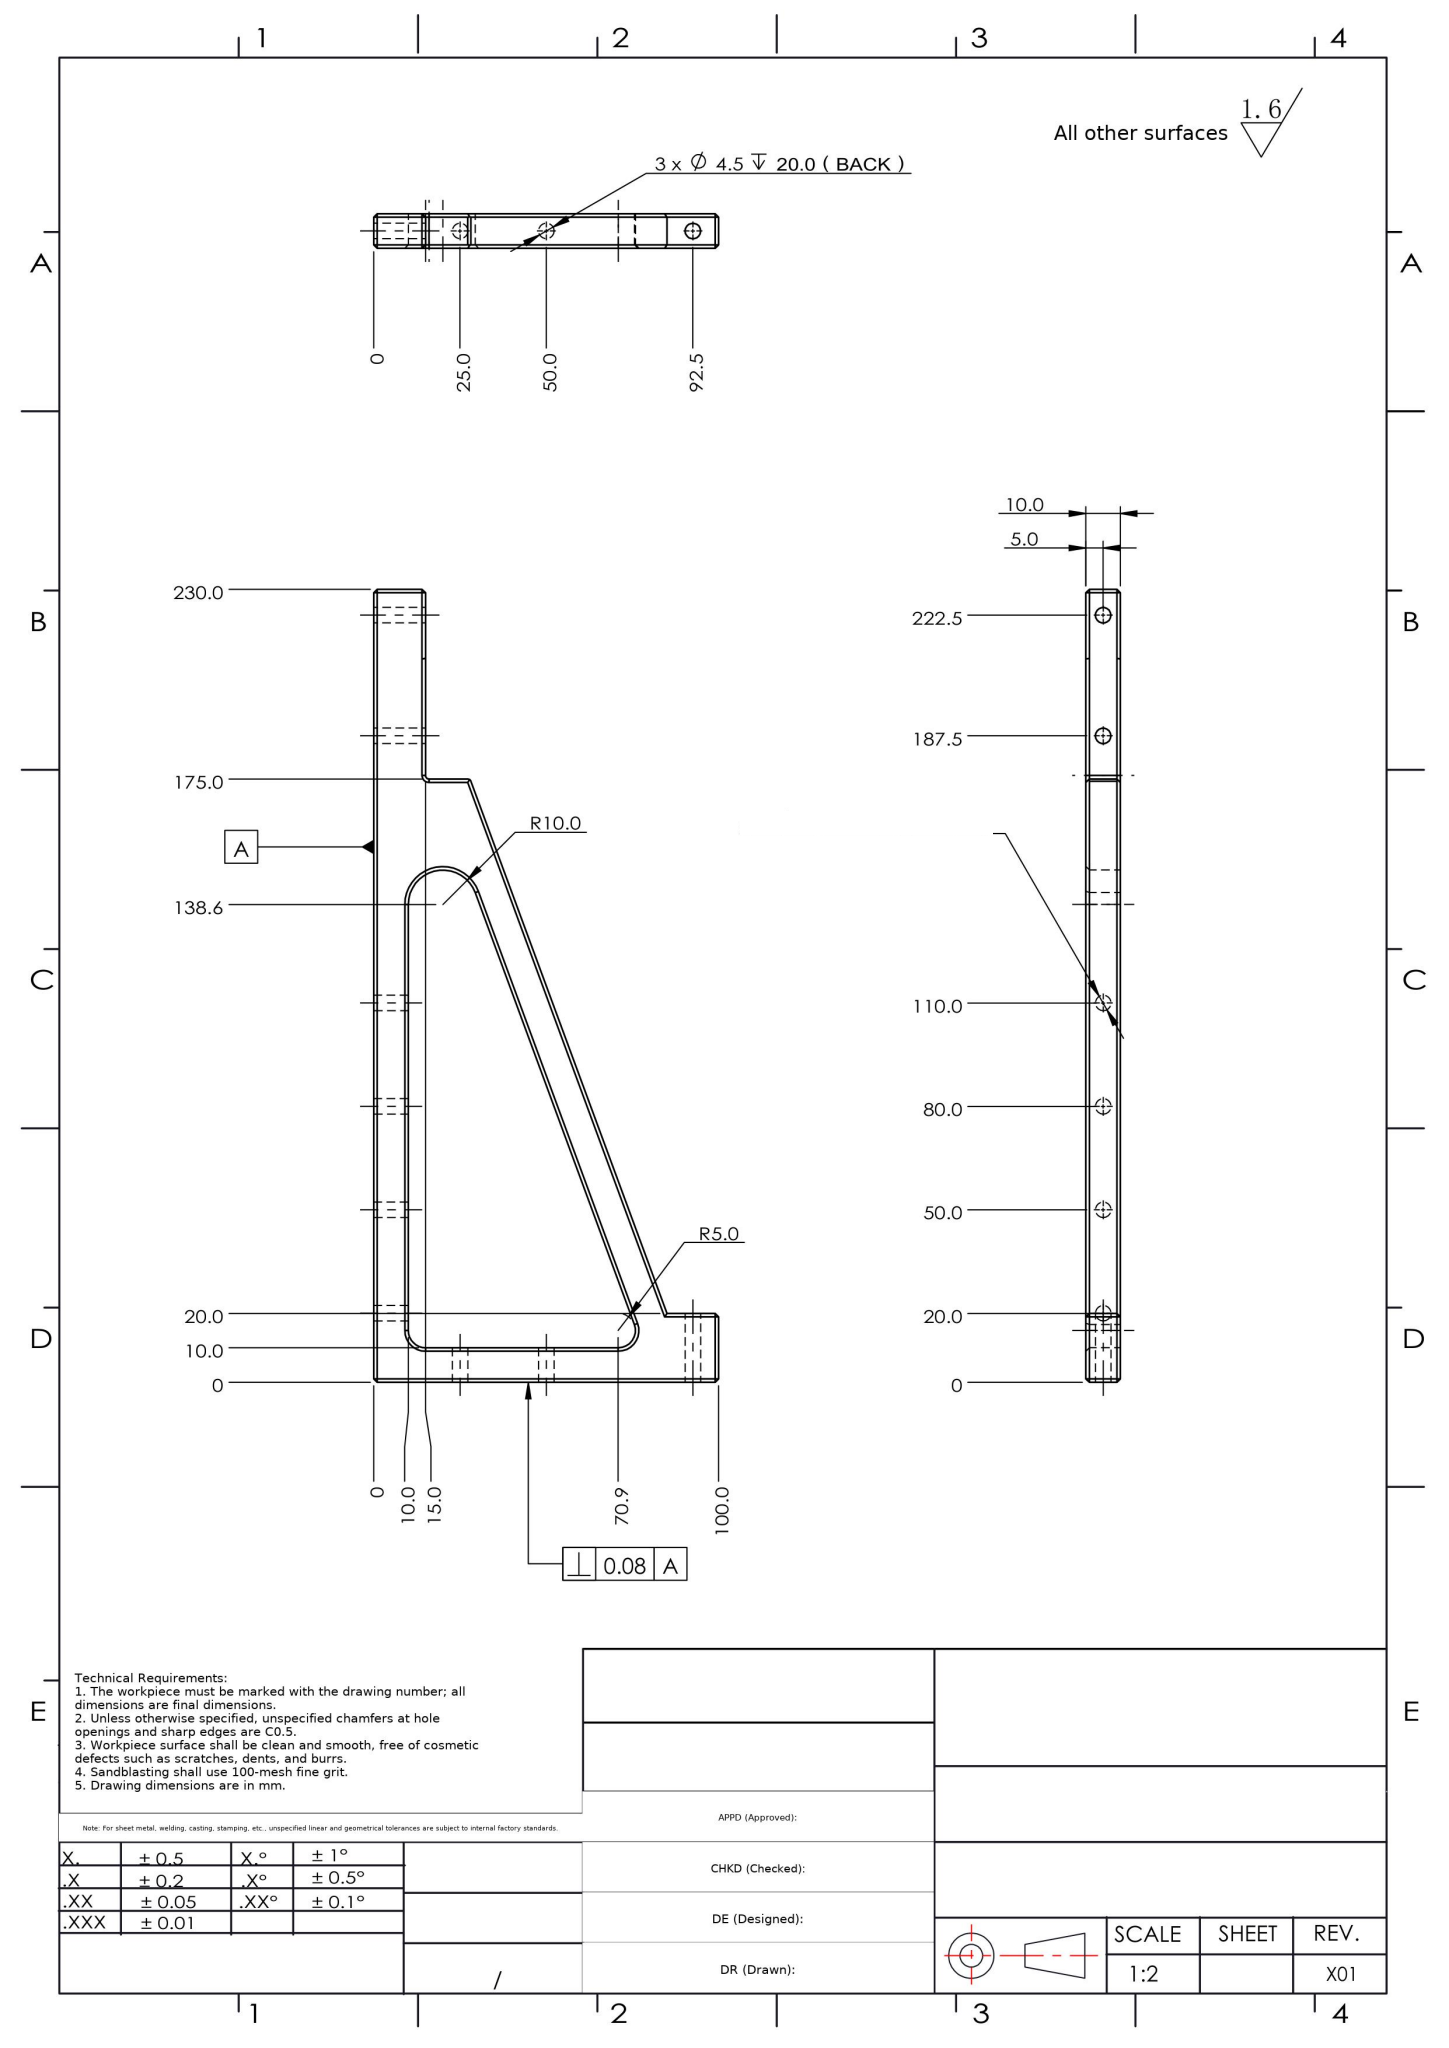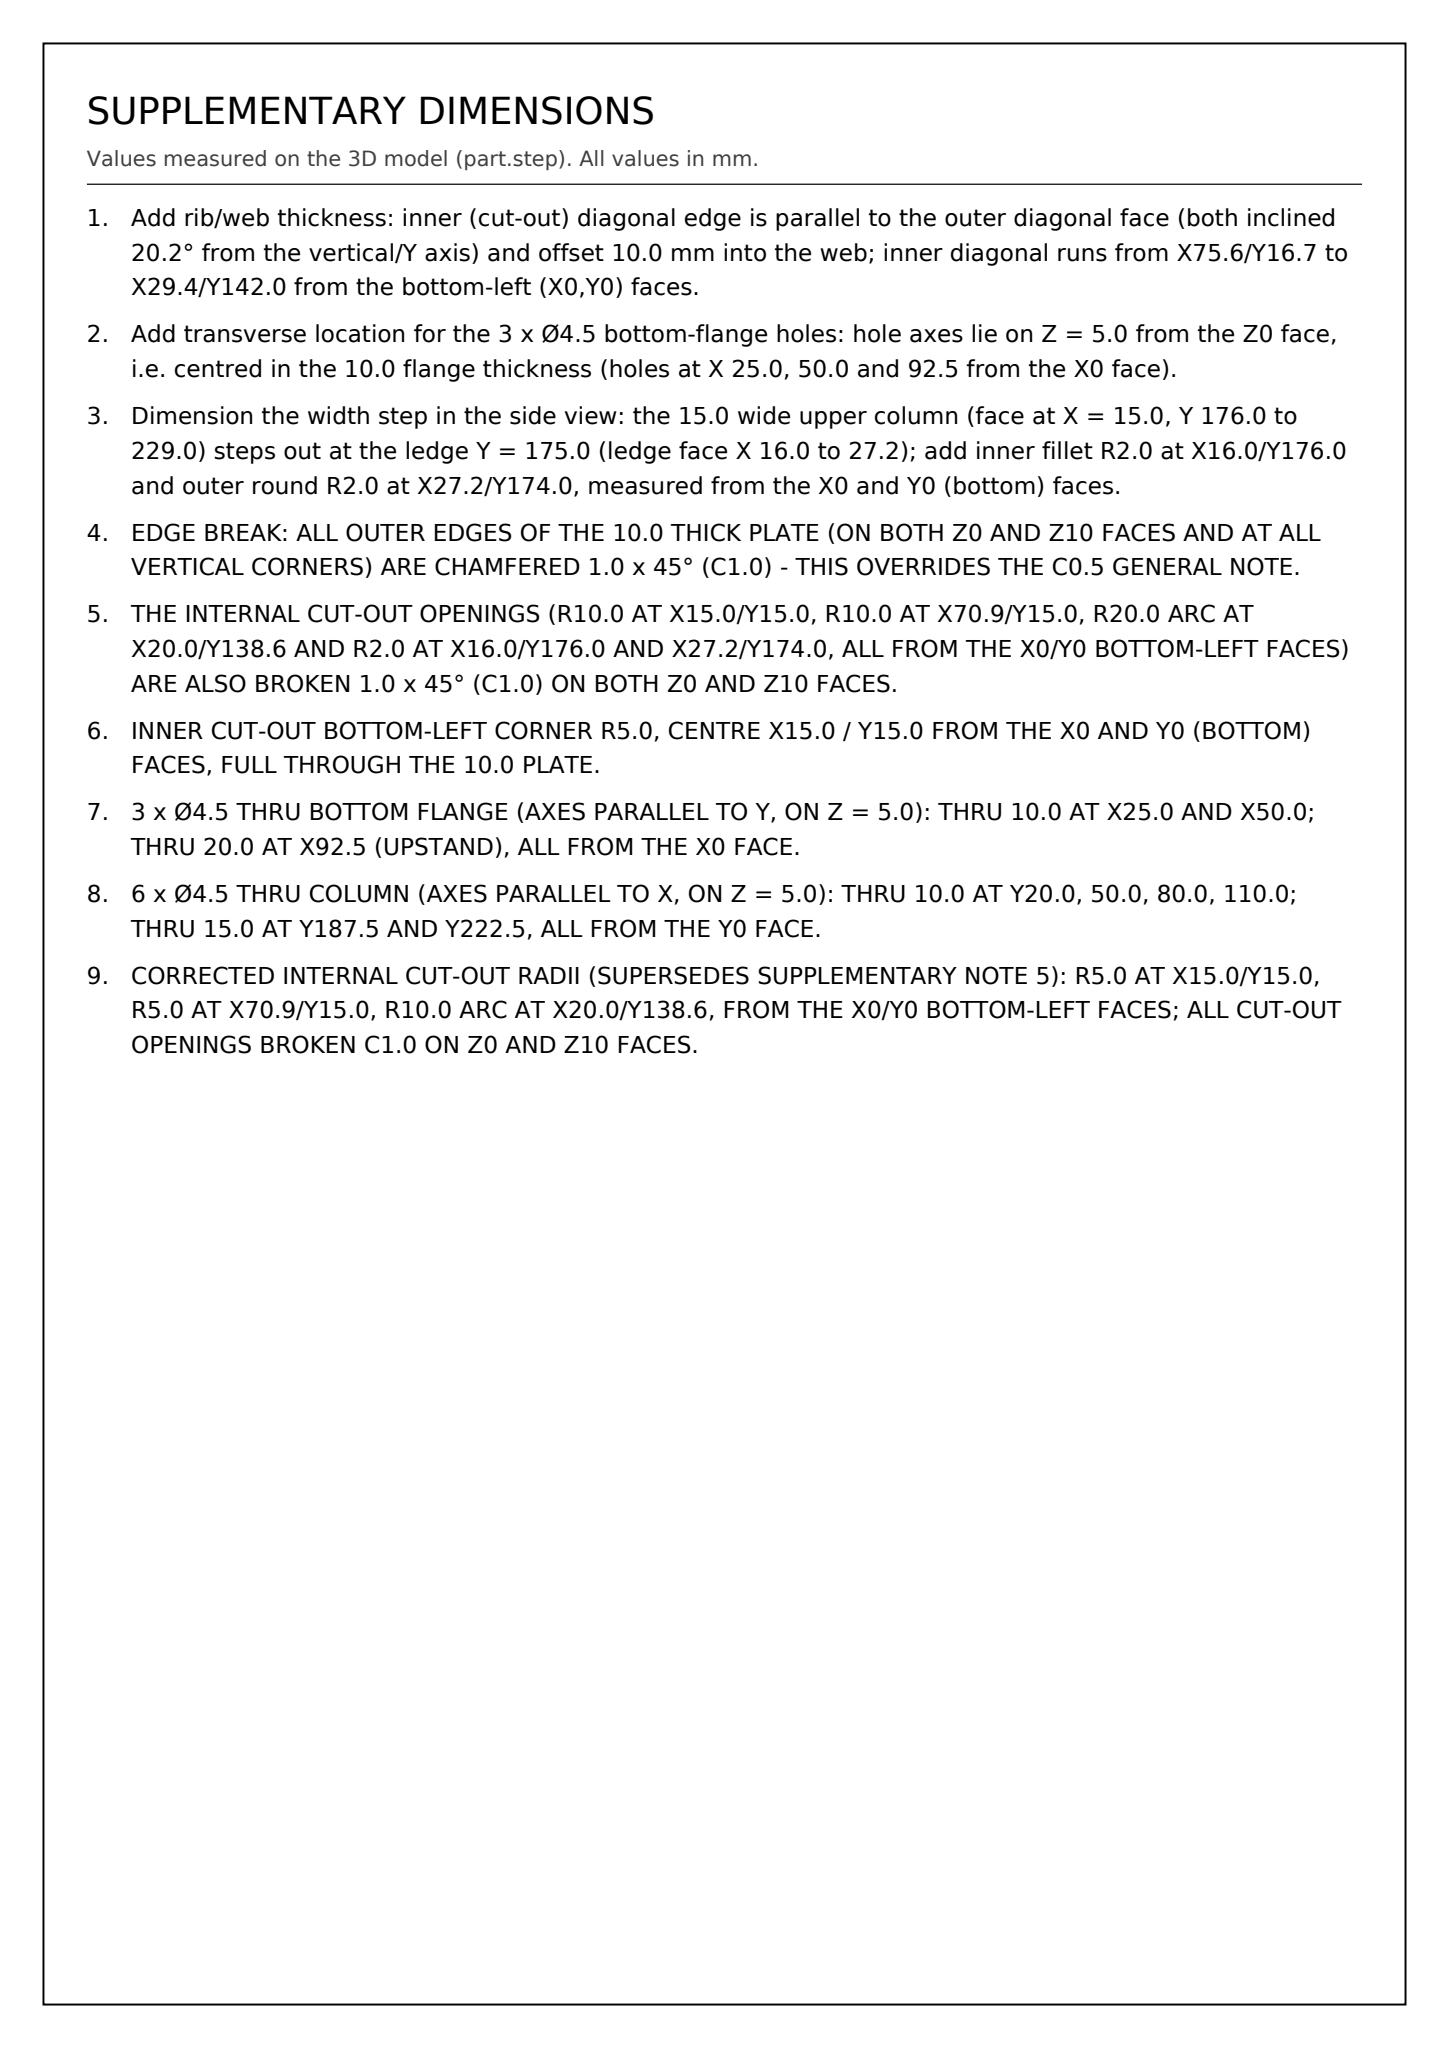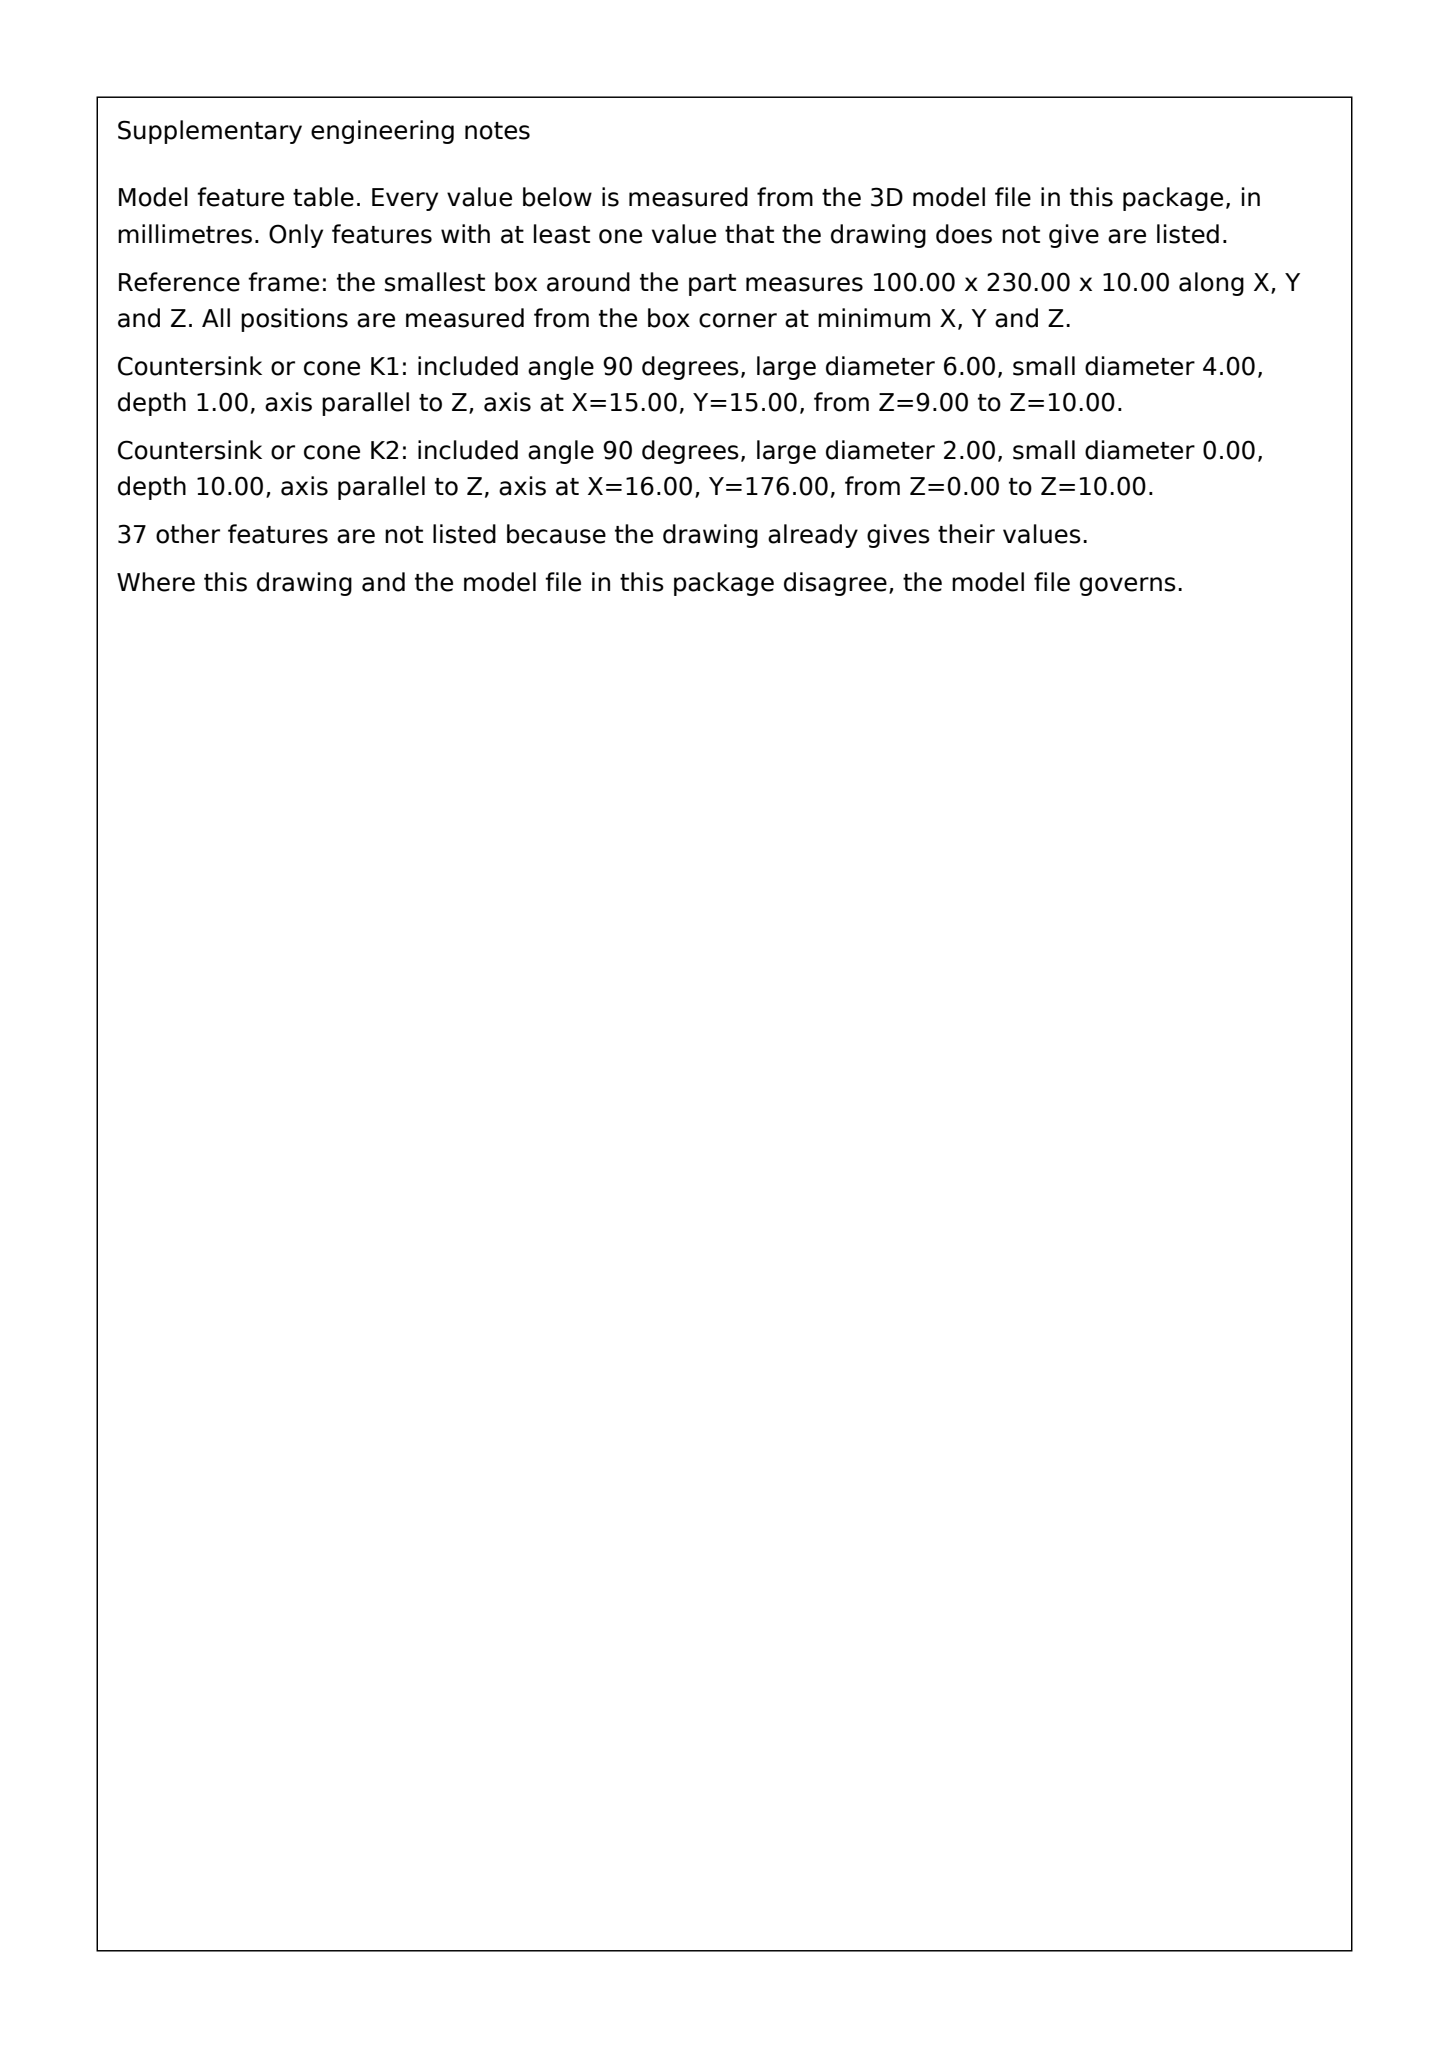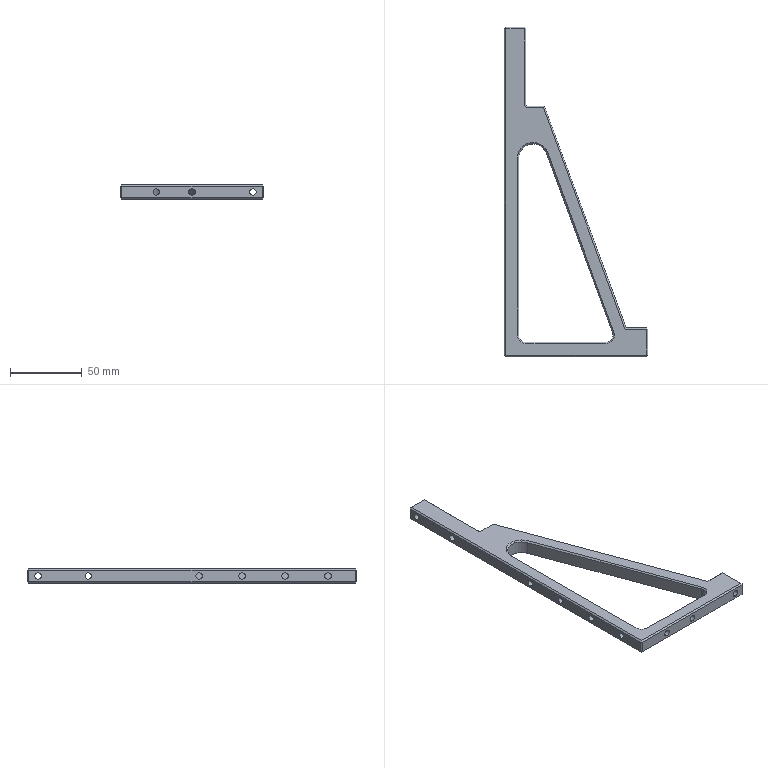Part | SolidWorks | mm | 1 solid | 79 faces | box 100 x 230 x 10 mm | volume 54764 mm3 | plane 49 | cylinder 24 | cone 6 | commonest cylinder face diameters 4.5 x18 10 x3 2 x2 20 x1
Drawing notes:
Add rib/web thickness: inner (cut-out) diagonal edge is parallel to the outer diagonal face (both inclined 20.2° from the vertical/Y axis) and offset 10.0 mm into the web; inner diagonal runs from X75.6/Y16.7 to X29.4/Y142.0 from the bottom-left (X0,Y0) faces. | from the solid: inclined_planes: two parallel faces with angle_to_xyz_axes [20.2,69.8,90.0] - outer bbox_from [28.1,20.0,1.0] size [56.9,154.3,8.0]; inner bbox_from [29.4,16.7,0.0] size [46.2,125.3,9.0] (perpendicular offset = 10.0)
Add transverse location for the 3 x Ø4.5 bottom-flange holes: hole axes lie on Z = 5.0 from the Z0 face, i.e. centred in the 10.0 flange thickness (holes at X 25.0, 50.0 and 92.5 from the X0 face). | from the solid: cylinders hole/bore Ø4.5 axis y at [25.0,null,5.0], [50.0,null,5.0], [92.5,null,5.0]
Dimension the width step in the side view: the 15.0 wide upper column (face at X = 15.0, Y 176.0 to 229.0) steps out at the ledge Y = 175.0 (ledge face X 16.0 to 27.2); add inner fillet R2.0 at X16.0/Y176.0 and outer round R2.0 at X27.2/Y174.0, measured from the X0 and Y0 (bottom) faces. | from the solid: axis_planes x=15.0 extent y[176.0,229.0]; y=175.0 extent x[16.0,27.2]; cylinders concave arc Ø2.0 at [16.0,176.0] and convex arc Ø2.0 at [27.2,174.0]
EDGE BREAK: ALL OUTER EDGES OF THE 10.0 THICK PLATE (ON BOTH Z0 AND Z10 FACES AND AT ALL VERTICAL CORNERS) ARE CHAMFERED 1.0 x 45° (C1.0) - THIS OVERRIDES THE C0.5 GENERAL NOTE. | from the solid: inclined_planes: 25 faces at 45°/45°/90° and 45°/90°/45° of 1.0 x 1.0 cross-section running along the periphery (e.g. bbox_from [0.0,1.0,0.0] size [1.0,228.0,1.0]; [99.0,1.0,9.0] size [1.0,18.0,1.0]; [0.0,0.0,1.0] size [1.0,1.0,8.0])
THE INTERNAL CUT-OUT OPENINGS (R10.0 AT X15.0/Y15.0, R10.0 AT X70.9/Y15.0, R20.0 ARC AT X20.0/Y138.6 AND R2.0 AT X16.0/Y176.0 AND X27.2/Y174.0, ALL FROM THE X0/Y0 BOTTOM-LEFT FACES) ARE ALSO BROKEN 1.0 x 45° (C1.0) ON BOTH Z0 AND Z10 FACES. | from the solid: cones: 90° included angle, 1.0 deep, at [9.0,9.0,9.0], [70.9,9.0,9.0], [9.0,138.6,9.0] (ref_dia 10.0/20.0) and ref_dia 4.0 at [14.0,174.0,0.0] and [14.0,174.0,9.0]; plus 45° inclined faces of 1.0 size along the inner diagonal (bbox_from [9.0,15.0,9.0] size [1.0,123.6,1.0], [29.4,16.7,9.0])
INNER CUT-OUT BOTTOM-LEFT CORNER R5.0, CENTRE X15.0 / Y15.0 FROM THE X0 AND Y0 (BOTTOM) FACES, FULL THROUGH THE 10.0 PLATE. | from the solid: cylinders: concave arc dia 10.0, axis z at [15.0, 15.0], z 0.0-9.0, 90 deg
3 x Ø4.5 THRU BOTTOM FLANGE (AXES PARALLEL TO Y, ON Z = 5.0): THRU 10.0 AT X25.0 AND X50.0; THRU 20.0 AT X92.5 (UPSTAND), ALL FROM THE X0 FACE. | from the solid: cylinders: hole/bore dia 4.5 axis y at x=25.0 and 50.0 (y 0.0-10.0) and x=92.5 (y 0.0-20.0), z=5.0
6 x Ø4.5 THRU COLUMN (AXES PARALLEL TO X, ON Z = 5.0): THRU 10.0 AT Y20.0, 50.0, 80.0, 110.0; THRU 15.0 AT Y187.5 AND Y222.5, ALL FROM THE Y0 FACE. | from the solid: cylinders: hole/bore dia 4.5 axis x at y=20.0/50.0/80.0/110.0 (x 0.0-10.0) and y=187.5/222.5 (x 0.0-15.0), z=5.0
CORRECTED INTERNAL CUT-OUT RADII (SUPERSEDES SUPPLEMENTARY NOTE 5): R5.0 AT X15.0/Y15.0, R5.0 AT X70.9/Y15.0, R10.0 ARC AT X20.0/Y138.6, FROM THE X0/Y0 BOTTOM-LEFT FACES; ALL CUT-OUT OPENINGS BROKEN C1.0 ON Z0 AND Z10 FACES. | from the solid: cylinders: concave arcs dia 10.0 at [15.0,15.0] and [70.9,15.0], dia 20.0 at [20.0,138.6]; cones 90 deg ref dia 10.0 / 20.0 at z 9.0-10.0